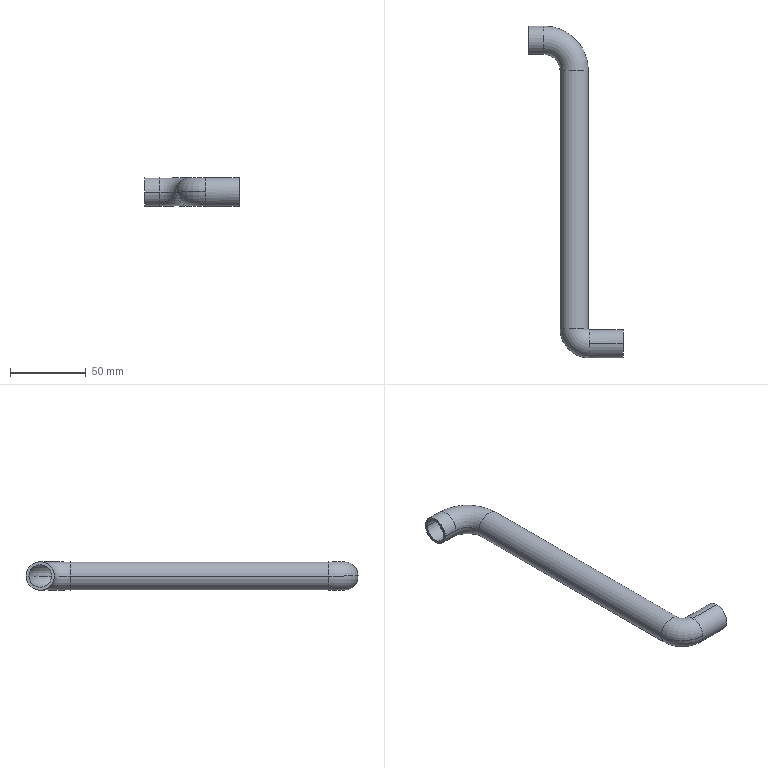Component | SolidWorks | PipeOne-1 | 1 solid | 22 faces | box 62.38 x 219.59 x 18.77 mm | volume 25031 mm3 | cylinder 12 | torus 8 | plane 2 | commonest cylinder face diameters 15 x6 18.77 x6
build123d program:
from build123d import *

# Parameters (mm, degrees)
SKETCH1_R   = 9.385
SKETCH1_R_2 = 7.5


with BuildPart() as part:
    # Sweep5: sweep along a path in Sketch3
    with BuildLine(Plane(origin=(0, 0, 0), x_dir=(0, 0, -1), z_dir=(1, 0, 0))) as sweep5_path:
        Line((0, 0), (-10, 0))
        ThreePointArc((-10, 0), (-24.142, -5.858), (-30, -20))
        Line((-30, -20), (-30, -190.823))
        ThreePointArc((-30, -190.823), (-32.929, -197.894), (-40, -200.823))
        Line((-40, -200.823), (-62.38, -200.823))
    # Sketch1 → Sweep5 (sweep)
    with BuildSketch(Plane.XY):
        Circle(SKETCH1_R)
        Circle(SKETCH1_R_2, mode=Mode.SUBTRACT)
    sweep(path=sweep5_path.line)


solid = part.part

# Placed as in the assembly
solid = solid.moved(Location((598.89, 510.198, -117.25), (0, 90, 0)))
STEP:
#1=CARTESIAN_POINT('',(25.055,12.574,-4.616));
#2=VERTEX_POINT('',#1);
#3=CARTESIAN_POINT('',(24.464,12.574,-4.616));
#4=VERTEX_POINT('',#3);
#5=CARTESIAN_POINT('',(24.759,12.574,-4.616));
#6=DIRECTION('',(-0.,1.,-0.));
#7=DIRECTION('',(0.,0.,-1.));
#8=AXIS2_PLACEMENT_3D('',#5,#6,#7);
#9=CIRCLE('',#8,0.2953);
#10=EDGE_CURVE('',#2,#4,#9,.T.);
#11=ORIENTED_EDGE('',*,*,#10,.T.);
#12=CARTESIAN_POINT('',(25.153,11.885,-4.616));
#13=VERTEX_POINT('',#12);
#14=CARTESIAN_POINT('',(25.153,12.574,-4.616));
#15=DIRECTION('',(-0.,0.,1.));
#16=DIRECTION('',(0.,-1.,0.));
#17=AXIS2_PLACEMENT_3D('',#14,#15,#16);
#18=CIRCLE('',#17,0.689);
#19=EDGE_CURVE('',#4,#13,#18,.T.);
#20=ORIENTED_EDGE('',*,*,#19,.T.);
#21=CARTESIAN_POINT('',(25.153,12.18,-4.911));
#22=VERTEX_POINT('',#21);
#23=CARTESIAN_POINT('',(25.153,12.18,-4.616));
#24=DIRECTION('',(-1.,-0.,-0.));
#25=DIRECTION('',(0.,-0.,-1.));
#26=AXIS2_PLACEMENT_3D('',#23,#24,#25);
#27=CIRCLE('',#26,0.2953);
#28=EDGE_CURVE('',#22,#13,#27,.T.);
#29=ORIENTED_EDGE('',*,*,#28,.F.);
#30=CARTESIAN_POINT('',(25.153,12.475,-4.616));
#31=VERTEX_POINT('',#30);
#32=CARTESIAN_POINT('',(25.153,12.18,-4.616));
#33=DIRECTION('',(-1.,-0.,-0.));
#34=DIRECTION('',(0.,-0.,-1.));
#35=AXIS2_PLACEMENT_3D('',#32,#33,#34);
#36=CIRCLE('',#35,0.2953);
#37=EDGE_CURVE('',#31,#22,#36,.T.);
#38=ORIENTED_EDGE('',*,*,#37,.F.);
#39=CARTESIAN_POINT('',(25.153,12.574,-4.616));
#40=DIRECTION('',(-0.,0.,1.));
#41=DIRECTION('',(0.,-1.,0.));
#42=AXIS2_PLACEMENT_3D('',#39,#40,#41);
#43=CIRCLE('',#42,0.09843);
#44=EDGE_CURVE('',#2,#31,#43,.T.);
#45=ORIENTED_EDGE('',*,*,#44,.F.);
#46=EDGE_LOOP('',(#11,#20,#29,#38,#45));
#47=FACE_OUTER_BOUND('',#46,.T.);
#48=CARTESIAN_POINT('',(25.153,12.574,-4.616));
#49=DIRECTION('',(-0.,0.,1.));
#50=DIRECTION('',(1.,0.,0.));
#51=AXIS2_PLACEMENT_3D('',#48,#49,#50);
#52=TOROIDAL_SURFACE('',#51,0.3937,0.2953);
#53=ADVANCED_FACE('',(#47),#52,.F.);
#54=CARTESIAN_POINT('',(23.972,19.791,-4.616));
#55=VERTEX_POINT('',#54);
#56=CARTESIAN_POINT('',(23.972,20.382,-4.616));
#57=VERTEX_POINT('',#56);
#58=CARTESIAN_POINT('',(23.972,20.087,-4.616));
#59=DIRECTION('',(-1.,-0.,-0.));
#60=DIRECTION('',(0.,0.,-1.));
#61=AXIS2_PLACEMENT_3D('',#58,#59,#60);
#62=CIRCLE('',#61,0.2953);
#63=EDGE_CURVE('',#55,#57,#62,.T.);
#64=ORIENTED_EDGE('',*,*,#63,.T.);
#65=CARTESIAN_POINT('',(25.055,19.299,-4.616));
#66=VERTEX_POINT('',#65);
#67=CARTESIAN_POINT('',(23.972,19.299,-4.616));
#68=DIRECTION('',(0.,-0.,-1.));
#69=DIRECTION('',(0.,1.,-0.));
#70=AXIS2_PLACEMENT_3D('',#67,#68,#69);
#71=CIRCLE('',#70,1.083);
#72=EDGE_CURVE('',#57,#66,#71,.T.);
#73=ORIENTED_EDGE('',*,*,#72,.T.);
#74=CARTESIAN_POINT('',(24.464,19.299,-4.616));
#75=VERTEX_POINT('',#74);
#76=CARTESIAN_POINT('',(24.759,19.299,-4.616));
#77=DIRECTION('',(-0.,1.,-0.));
#78=DIRECTION('',(0.,0.,-1.));
#79=AXIS2_PLACEMENT_3D('',#76,#77,#78);
#80=CIRCLE('',#79,0.2953);
#81=EDGE_CURVE('',#75,#66,#80,.T.);
#82=ORIENTED_EDGE('',*,*,#81,.F.);
#83=CARTESIAN_POINT('',(23.972,19.299,-4.616));
#84=DIRECTION('',(0.,-0.,-1.));
#85=DIRECTION('',(0.,1.,-0.));
#86=AXIS2_PLACEMENT_3D('',#83,#84,#85);
#87=CIRCLE('',#86,0.4921);
#88=EDGE_CURVE('',#55,#75,#87,.T.);
#89=ORIENTED_EDGE('',*,*,#88,.F.);
#90=EDGE_LOOP('',(#64,#73,#82,#89));
#91=FACE_OUTER_BOUND('',#90,.T.);
#92=CARTESIAN_POINT('',(23.972,19.299,-4.616));
#93=DIRECTION('',(0.,-0.,-1.));
#94=DIRECTION('',(-1.,-0.,-0.));
#95=AXIS2_PLACEMENT_3D('',#92,#93,#94);
#96=TOROIDAL_SURFACE('',#95,0.7874,0.2953);
#97=ADVANCED_FACE('',(#91),#96,.F.);
#98=CARTESIAN_POINT('',(25.129,12.574,-4.616));
#99=VERTEX_POINT('',#98);
#100=CARTESIAN_POINT('',(24.39,12.574,-4.616));
#101=VERTEX_POINT('',#100);
#102=CARTESIAN_POINT('',(24.759,12.574,-4.616));
#103=DIRECTION('',(0.,-1.,0.));
#104=DIRECTION('',(0.,-0.,-1.));
#105=AXIS2_PLACEMENT_3D('',#102,#103,#104);
#106=CIRCLE('',#105,0.3695);
#107=EDGE_CURVE('',#99,#101,#106,.T.);
#108=ORIENTED_EDGE('',*,*,#107,.T.);
#109=CARTESIAN_POINT('',(25.153,11.811,-4.616));
#110=VERTEX_POINT('',#109);
#111=CARTESIAN_POINT('',(25.153,12.574,-4.616));
#112=DIRECTION('',(-0.,0.,1.));
#113=DIRECTION('',(0.,-1.,0.));
#114=AXIS2_PLACEMENT_3D('',#111,#112,#113);
#115=CIRCLE('',#114,0.7632);
#116=EDGE_CURVE('',#101,#110,#115,.T.);
#117=ORIENTED_EDGE('',*,*,#116,.T.);
#118=CARTESIAN_POINT('',(25.153,12.18,-4.247));
#119=VERTEX_POINT('',#118);
#120=CARTESIAN_POINT('',(25.153,12.18,-4.616));
#121=DIRECTION('',(1.,0.,0.));
#122=DIRECTION('',(0.,-0.,-1.));
#123=AXIS2_PLACEMENT_3D('',#120,#121,#122);
#124=CIRCLE('',#123,0.3695);
#125=EDGE_CURVE('',#119,#110,#124,.T.);
#126=ORIENTED_EDGE('',*,*,#125,.F.);
#127=CARTESIAN_POINT('',(25.153,12.55,-4.616));
#128=VERTEX_POINT('',#127);
#129=CARTESIAN_POINT('',(25.153,12.18,-4.616));
#130=DIRECTION('',(1.,0.,0.));
#131=DIRECTION('',(0.,-0.,-1.));
#132=AXIS2_PLACEMENT_3D('',#129,#130,#131);
#133=CIRCLE('',#132,0.3695);
#134=EDGE_CURVE('',#128,#119,#133,.T.);
#135=ORIENTED_EDGE('',*,*,#134,.F.);
#136=CARTESIAN_POINT('',(25.153,12.574,-4.616));
#137=DIRECTION('',(-0.,0.,1.));
#138=DIRECTION('',(0.,-1.,0.));
#139=AXIS2_PLACEMENT_3D('',#136,#137,#138);
#140=CIRCLE('',#139,0.02421);
#141=EDGE_CURVE('',#99,#128,#140,.T.);
#142=ORIENTED_EDGE('',*,*,#141,.F.);
#143=EDGE_LOOP('',(#108,#117,#126,#135,#142));
#144=FACE_OUTER_BOUND('',#143,.T.);
#145=CARTESIAN_POINT('',(25.153,12.574,-4.616));
#146=DIRECTION('',(-0.,0.,1.));
#147=DIRECTION('',(1.,0.,0.));
#148=AXIS2_PLACEMENT_3D('',#145,#146,#147);
#149=TOROIDAL_SURFACE('',#148,0.3937,0.3695);
#150=ADVANCED_FACE('',(#144),#149,.T.);
#151=CARTESIAN_POINT('',(23.972,19.717,-4.616));
#152=VERTEX_POINT('',#151);
#153=CARTESIAN_POINT('',(23.972,20.456,-4.616));
#154=VERTEX_POINT('',#153);
#155=CARTESIAN_POINT('',(23.972,20.087,-4.616));
#156=DIRECTION('',(1.,0.,0.));
#157=DIRECTION('',(0.,0.,-1.));
#158=AXIS2_PLACEMENT_3D('',#155,#156,#157);
#159=CIRCLE('',#158,0.3695);
#160=EDGE_CURVE('',#152,#154,#159,.T.);
#161=ORIENTED_EDGE('',*,*,#160,.T.);
#162=CARTESIAN_POINT('',(25.129,19.299,-4.616));
#163=VERTEX_POINT('',#162);
#164=CARTESIAN_POINT('',(23.972,19.299,-4.616));
#165=DIRECTION('',(0.,-0.,-1.));
#166=DIRECTION('',(0.,1.,-0.));
#167=AXIS2_PLACEMENT_3D('',#164,#165,#166);
#168=CIRCLE('',#167,1.157);
#169=EDGE_CURVE('',#154,#163,#168,.T.);
#170=ORIENTED_EDGE('',*,*,#169,.T.);
#171=CARTESIAN_POINT('',(24.39,19.299,-4.616));
#172=VERTEX_POINT('',#171);
#173=CARTESIAN_POINT('',(24.759,19.299,-4.616));
#174=DIRECTION('',(0.,-1.,0.));
#175=DIRECTION('',(0.,-0.,-1.));
#176=AXIS2_PLACEMENT_3D('',#173,#174,#175);
#177=CIRCLE('',#176,0.3695);
#178=EDGE_CURVE('',#172,#163,#177,.T.);
#179=ORIENTED_EDGE('',*,*,#178,.F.);
#180=CARTESIAN_POINT('',(23.972,19.299,-4.616));
#181=DIRECTION('',(0.,-0.,-1.));
#182=DIRECTION('',(0.,1.,-0.));
#183=AXIS2_PLACEMENT_3D('',#180,#181,#182);
#184=CIRCLE('',#183,0.4179);
#185=EDGE_CURVE('',#152,#172,#184,.T.);
#186=ORIENTED_EDGE('',*,*,#185,.F.);
#187=EDGE_LOOP('',(#161,#170,#179,#186));
#188=FACE_OUTER_BOUND('',#187,.T.);
#189=CARTESIAN_POINT('',(23.972,19.299,-4.616));
#190=DIRECTION('',(0.,-0.,-1.));
#191=DIRECTION('',(-1.,-0.,-0.));
#192=AXIS2_PLACEMENT_3D('',#189,#190,#191);
#193=TOROIDAL_SURFACE('',#192,0.7874,0.3695);
#194=ADVANCED_FACE('',(#188),#193,.T.);
#195=ORIENTED_EDGE('',*,*,#28,.T.);
#196=CARTESIAN_POINT('',(25.153,12.18,-4.321));
#197=VERTEX_POINT('',#196);
#198=CARTESIAN_POINT('',(25.153,12.18,-4.616));
#199=DIRECTION('',(-1.,-0.,-0.));
#200=DIRECTION('',(0.,0.,-1.));
#201=AXIS2_PLACEMENT_3D('',#198,#199,#200);
#202=CIRCLE('',#201,0.2953);
#203=EDGE_CURVE('',#13,#197,#202,.T.);
#204=ORIENTED_EDGE('',*,*,#203,.T.);
#205=CARTESIAN_POINT('',(26.034,12.18,-4.321));
#206=VERTEX_POINT('',#205);
#207=CARTESIAN_POINT('',(25.153,12.18,-4.321));
#208=DIRECTION('',(1.,0.,0.));
#209=VECTOR('',#208,39.37);
#210=LINE('',#207,#209);
#211=EDGE_CURVE('',#197,#206,#210,.T.);
#212=ORIENTED_EDGE('',*,*,#211,.T.);
#213=CARTESIAN_POINT('',(26.034,12.18,-4.911));
#214=VERTEX_POINT('',#213);
#215=CARTESIAN_POINT('',(26.034,12.18,-4.616));
#216=DIRECTION('',(-1.,-0.,-0.));
#217=DIRECTION('',(0.,-0.,-1.));
#218=AXIS2_PLACEMENT_3D('',#215,#216,#217);
#219=CIRCLE('',#218,0.2953);
#220=EDGE_CURVE('',#214,#206,#219,.T.);
#221=ORIENTED_EDGE('',*,*,#220,.F.);
#222=CARTESIAN_POINT('',(25.153,12.18,-4.911));
#223=DIRECTION('',(1.,0.,0.));
#224=VECTOR('',#223,39.37);
#225=LINE('',#222,#224);
#226=EDGE_CURVE('',#22,#214,#225,.T.);
#227=ORIENTED_EDGE('',*,*,#226,.F.);
#228=EDGE_LOOP('',(#195,#204,#212,#221,#227));
#229=FACE_OUTER_BOUND('',#228,.T.);
#230=CARTESIAN_POINT('',(25.153,12.18,-4.616));
#231=DIRECTION('',(1.,0.,0.));
#232=DIRECTION('',(0.,0.,-1.));
#233=AXIS2_PLACEMENT_3D('',#230,#231,#232);
#234=CYLINDRICAL_SURFACE('',#233,0.2953);
#235=ADVANCED_FACE('',(#229),#234,.F.);
#236=ORIENTED_EDGE('',*,*,#81,.T.);
#237=CARTESIAN_POINT('',(25.055,19.299,-4.616));
#238=DIRECTION('',(0.,-1.,0.));
#239=VECTOR('',#238,39.37);
#240=LINE('',#237,#239);
#241=EDGE_CURVE('',#66,#2,#240,.T.);
#242=ORIENTED_EDGE('',*,*,#241,.T.);
#243=CARTESIAN_POINT('',(24.759,12.574,-4.616));
#244=DIRECTION('',(-0.,1.,-0.));
#245=DIRECTION('',(0.,0.,-1.));
#246=AXIS2_PLACEMENT_3D('',#243,#244,#245);
#247=CIRCLE('',#246,0.2953);
#248=EDGE_CURVE('',#4,#2,#247,.T.);
#249=ORIENTED_EDGE('',*,*,#248,.F.);
#250=CARTESIAN_POINT('',(24.464,19.299,-4.616));
#251=DIRECTION('',(0.,-1.,0.));
#252=VECTOR('',#251,39.37);
#253=LINE('',#250,#252);
#254=EDGE_CURVE('',#75,#4,#253,.T.);
#255=ORIENTED_EDGE('',*,*,#254,.F.);
#256=EDGE_LOOP('',(#236,#242,#249,#255));
#257=FACE_OUTER_BOUND('',#256,.T.);
#258=CARTESIAN_POINT('',(24.759,19.299,-4.616));
#259=DIRECTION('',(0.,-1.,0.));
#260=DIRECTION('',(-1.,0.,0.));
#261=AXIS2_PLACEMENT_3D('',#258,#259,#260);
#262=CYLINDRICAL_SURFACE('',#261,0.2953);
#263=ADVANCED_FACE('',(#257),#262,.F.);
#264=CARTESIAN_POINT('',(23.578,19.791,-4.616));
#265=VERTEX_POINT('',#264);
#266=CARTESIAN_POINT('',(23.578,20.382,-4.616));
#267=VERTEX_POINT('',#266);
#268=CARTESIAN_POINT('',(23.578,20.087,-4.616));
#269=DIRECTION('',(-1.,-0.,-0.));
#270=DIRECTION('',(0.,0.,-1.));
#271=AXIS2_PLACEMENT_3D('',#268,#269,#270);
#272=CIRCLE('',#271,0.2953);
#273=EDGE_CURVE('',#265,#267,#272,.T.);
#274=ORIENTED_EDGE('',*,*,#273,.T.);
#275=CARTESIAN_POINT('',(23.578,20.382,-4.616));
#276=DIRECTION('',(1.,0.,0.));
#277=VECTOR('',#276,39.37);
#278=LINE('',#275,#277);
#279=EDGE_CURVE('',#267,#57,#278,.T.);
#280=ORIENTED_EDGE('',*,*,#279,.T.);
#281=ORIENTED_EDGE('',*,*,#63,.F.);
#282=CARTESIAN_POINT('',(23.578,19.791,-4.616));
#283=DIRECTION('',(1.,0.,0.));
#284=VECTOR('',#283,39.37);
#285=LINE('',#282,#284);
#286=EDGE_CURVE('',#265,#55,#285,.T.);
#287=ORIENTED_EDGE('',*,*,#286,.F.);
#288=EDGE_LOOP('',(#274,#280,#281,#287));
#289=FACE_OUTER_BOUND('',#288,.T.);
#290=CARTESIAN_POINT('',(23.578,20.087,-4.616));
#291=DIRECTION('',(1.,0.,0.));
#292=DIRECTION('',(0.,-1.,0.));
#293=AXIS2_PLACEMENT_3D('',#290,#291,#292);
#294=CYLINDRICAL_SURFACE('',#293,0.2953);
#295=ADVANCED_FACE('',(#289),#294,.F.);
#296=CARTESIAN_POINT('',(25.153,12.18,-4.986));
#297=VERTEX_POINT('',#296);
#298=CARTESIAN_POINT('',(25.153,12.18,-4.616));
#299=DIRECTION('',(1.,0.,0.));
#300=DIRECTION('',(0.,-0.,-1.));
#301=AXIS2_PLACEMENT_3D('',#298,#299,#300);
#302=CIRCLE('',#301,0.3695);
#303=EDGE_CURVE('',#297,#128,#302,.T.);
#304=ORIENTED_EDGE('',*,*,#303,.T.);
#305=ORIENTED_EDGE('',*,*,#134,.T.);
#306=CARTESIAN_POINT('',(26.034,12.18,-4.247));
#307=VERTEX_POINT('',#306);
#308=CARTESIAN_POINT('',(25.153,12.18,-4.247));
#309=DIRECTION('',(1.,0.,0.));
#310=VECTOR('',#309,39.37);
#311=LINE('',#308,#310);
#312=EDGE_CURVE('',#119,#307,#311,.T.);
#313=ORIENTED_EDGE('',*,*,#312,.T.);
#314=CARTESIAN_POINT('',(26.034,12.18,-4.986));
#315=VERTEX_POINT('',#314);
#316=CARTESIAN_POINT('',(26.034,12.18,-4.616));
#317=DIRECTION('',(1.,0.,0.));
#318=DIRECTION('',(0.,-0.,-1.));
#319=AXIS2_PLACEMENT_3D('',#316,#317,#318);
#320=CIRCLE('',#319,0.3695);
#321=EDGE_CURVE('',#315,#307,#320,.T.);
#322=ORIENTED_EDGE('',*,*,#321,.F.);
#323=CARTESIAN_POINT('',(25.153,12.18,-4.986));
#324=DIRECTION('',(1.,0.,0.));
#325=VECTOR('',#324,39.37);
#326=LINE('',#323,#325);
#327=EDGE_CURVE('',#297,#315,#326,.T.);
#328=ORIENTED_EDGE('',*,*,#327,.F.);
#329=EDGE_LOOP('',(#304,#305,#313,#322,#328));
#330=FACE_OUTER_BOUND('',#329,.T.);
#331=CARTESIAN_POINT('',(25.153,12.18,-4.616));
#332=DIRECTION('',(1.,0.,0.));
#333=DIRECTION('',(0.,-0.,-1.));
#334=AXIS2_PLACEMENT_3D('',#331,#332,#333);
#335=CYLINDRICAL_SURFACE('',#334,0.3695);
#336=ADVANCED_FACE('',(#330),#335,.T.);
#337=ORIENTED_EDGE('',*,*,#178,.T.);
#338=CARTESIAN_POINT('',(25.129,19.299,-4.616));
#339=DIRECTION('',(0.,-1.,0.));
#340=VECTOR('',#339,39.37);
#341=LINE('',#338,#340);
#342=EDGE_CURVE('',#163,#99,#341,.T.);
#343=ORIENTED_EDGE('',*,*,#342,.T.);
#344=CARTESIAN_POINT('',(24.759,12.574,-4.616));
#345=DIRECTION('',(0.,-1.,0.));
#346=DIRECTION('',(0.,-0.,-1.));
#347=AXIS2_PLACEMENT_3D('',#344,#345,#346);
#348=CIRCLE('',#347,0.3695);
#349=EDGE_CURVE('',#101,#99,#348,.T.);
#350=ORIENTED_EDGE('',*,*,#349,.F.);
#351=CARTESIAN_POINT('',(24.39,19.299,-4.616));
#352=DIRECTION('',(0.,-1.,0.));
#353=VECTOR('',#352,39.37);
#354=LINE('',#351,#353);
#355=EDGE_CURVE('',#172,#101,#354,.T.);
#356=ORIENTED_EDGE('',*,*,#355,.F.);
#357=EDGE_LOOP('',(#337,#343,#350,#356));
#358=FACE_OUTER_BOUND('',#357,.T.);
#359=CARTESIAN_POINT('',(24.759,19.299,-4.616));
#360=DIRECTION('',(0.,-1.,0.));
#361=DIRECTION('',(-1.,-0.,0.));
#362=AXIS2_PLACEMENT_3D('',#359,#360,#361);
#363=CYLINDRICAL_SURFACE('',#362,0.3695);
#364=ADVANCED_FACE('',(#358),#363,.T.);
#365=CARTESIAN_POINT('',(23.578,19.717,-4.616));
#366=VERTEX_POINT('',#365);
#367=CARTESIAN_POINT('',(23.578,20.456,-4.616));
#368=VERTEX_POINT('',#367);
#369=CARTESIAN_POINT('',(23.578,20.087,-4.616));
#370=DIRECTION('',(1.,0.,0.));
#371=DIRECTION('',(0.,0.,-1.));
#372=AXIS2_PLACEMENT_3D('',#369,#370,#371);
#373=CIRCLE('',#372,0.3695);
#374=EDGE_CURVE('',#366,#368,#373,.T.);
#375=ORIENTED_EDGE('',*,*,#374,.T.);
#376=CARTESIAN_POINT('',(23.578,20.456,-4.616));
#377=DIRECTION('',(1.,0.,0.));
#378=VECTOR('',#377,39.37);
#379=LINE('',#376,#378);
#380=EDGE_CURVE('',#368,#154,#379,.T.);
#381=ORIENTED_EDGE('',*,*,#380,.T.);
#382=ORIENTED_EDGE('',*,*,#160,.F.);
#383=CARTESIAN_POINT('',(23.578,19.717,-4.616));
#384=DIRECTION('',(1.,0.,0.));
#385=VECTOR('',#384,39.37);
#386=LINE('',#383,#385);
#387=EDGE_CURVE('',#366,#152,#386,.T.);
#388=ORIENTED_EDGE('',*,*,#387,.F.);
#389=EDGE_LOOP('',(#375,#381,#382,#388));
#390=FACE_OUTER_BOUND('',#389,.T.);
#391=CARTESIAN_POINT('',(23.578,20.087,-4.616));
#392=DIRECTION('',(1.,0.,0.));
#393=DIRECTION('',(0.,-1.,0.));
#394=AXIS2_PLACEMENT_3D('',#391,#392,#393);
#395=CYLINDRICAL_SURFACE('',#394,0.3695);
#396=ADVANCED_FACE('',(#390),#395,.T.);
#397=ORIENTED_EDGE('',*,*,#211,.F.);
#398=CARTESIAN_POINT('',(25.153,12.18,-4.616));
#399=DIRECTION('',(-1.,-0.,-0.));
#400=DIRECTION('',(0.,0.,-1.));
#401=AXIS2_PLACEMENT_3D('',#398,#399,#400);
#402=CIRCLE('',#401,0.2953);
#403=EDGE_CURVE('',#197,#31,#402,.T.);
#404=ORIENTED_EDGE('',*,*,#403,.T.);
#405=ORIENTED_EDGE('',*,*,#37,.T.);
#406=ORIENTED_EDGE('',*,*,#226,.T.);
#407=CARTESIAN_POINT('',(26.034,12.18,-4.616));
#408=DIRECTION('',(-1.,-0.,-0.));
#409=DIRECTION('',(0.,-0.,-1.));
#410=AXIS2_PLACEMENT_3D('',#407,#408,#409);
#411=CIRCLE('',#410,0.2953);
#412=EDGE_CURVE('',#206,#214,#411,.T.);
#413=ORIENTED_EDGE('',*,*,#412,.F.);
#414=EDGE_LOOP('',(#397,#404,#405,#406,#413));
#415=FACE_OUTER_BOUND('',#414,.T.);
#416=CARTESIAN_POINT('',(25.153,12.18,-4.616));
#417=DIRECTION('',(1.,0.,0.));
#418=DIRECTION('',(0.,0.,-1.));
#419=AXIS2_PLACEMENT_3D('',#416,#417,#418);
#420=CYLINDRICAL_SURFACE('',#419,0.2953);
#421=ADVANCED_FACE('',(#415),#420,.F.);
#422=ORIENTED_EDGE('',*,*,#19,.F.);
#423=ORIENTED_EDGE('',*,*,#248,.T.);
#424=ORIENTED_EDGE('',*,*,#44,.T.);
#425=ORIENTED_EDGE('',*,*,#403,.F.);
#426=ORIENTED_EDGE('',*,*,#203,.F.);
#427=EDGE_LOOP('',(#422,#423,#424,#425,#426));
#428=FACE_OUTER_BOUND('',#427,.T.);
#429=CARTESIAN_POINT('',(25.153,12.574,-4.616));
#430=DIRECTION('',(-0.,0.,1.));
#431=DIRECTION('',(1.,0.,0.));
#432=AXIS2_PLACEMENT_3D('',#429,#430,#431);
#433=TOROIDAL_SURFACE('',#432,0.3937,0.2953);
#434=ADVANCED_FACE('',(#428),#433,.F.);
#435=ORIENTED_EDGE('',*,*,#241,.F.);
#436=CARTESIAN_POINT('',(24.759,19.299,-4.616));
#437=DIRECTION('',(-0.,1.,-0.));
#438=DIRECTION('',(0.,0.,-1.));
#439=AXIS2_PLACEMENT_3D('',#436,#437,#438);
#440=CIRCLE('',#439,0.2953);
#441=EDGE_CURVE('',#66,#75,#440,.T.);
#442=ORIENTED_EDGE('',*,*,#441,.T.);
#443=ORIENTED_EDGE('',*,*,#254,.T.);
#444=ORIENTED_EDGE('',*,*,#10,.F.);
#445=EDGE_LOOP('',(#435,#442,#443,#444));
#446=FACE_OUTER_BOUND('',#445,.T.);
#447=CARTESIAN_POINT('',(24.759,19.299,-4.616));
#448=DIRECTION('',(0.,-1.,0.));
#449=DIRECTION('',(-1.,0.,0.));
#450=AXIS2_PLACEMENT_3D('',#447,#448,#449);
#451=CYLINDRICAL_SURFACE('',#450,0.2953);
#452=ADVANCED_FACE('',(#446),#451,.F.);
#453=ORIENTED_EDGE('',*,*,#72,.F.);
#454=CARTESIAN_POINT('',(23.972,20.087,-4.616));
#455=DIRECTION('',(-1.,-0.,-0.));
#456=DIRECTION('',(0.,0.,-1.));
#457=AXIS2_PLACEMENT_3D('',#454,#455,#456);
#458=CIRCLE('',#457,0.2953);
#459=EDGE_CURVE('',#57,#55,#458,.T.);
#460=ORIENTED_EDGE('',*,*,#459,.T.);
#461=ORIENTED_EDGE('',*,*,#88,.T.);
#462=ORIENTED_EDGE('',*,*,#441,.F.);
#463=EDGE_LOOP('',(#453,#460,#461,#462));
#464=FACE_OUTER_BOUND('',#463,.T.);
#465=CARTESIAN_POINT('',(23.972,19.299,-4.616));
#466=DIRECTION('',(0.,-0.,-1.));
#467=DIRECTION('',(-1.,-0.,-0.));
#468=AXIS2_PLACEMENT_3D('',#465,#466,#467);
#469=TOROIDAL_SURFACE('',#468,0.7874,0.2953);
#470=ADVANCED_FACE('',(#464),#469,.F.);
#471=ORIENTED_EDGE('',*,*,#279,.F.);
#472=CARTESIAN_POINT('',(23.578,20.087,-4.616));
#473=DIRECTION('',(-1.,-0.,-0.));
#474=DIRECTION('',(0.,0.,-1.));
#475=AXIS2_PLACEMENT_3D('',#472,#473,#474);
#476=CIRCLE('',#475,0.2953);
#477=EDGE_CURVE('',#267,#265,#476,.T.);
#478=ORIENTED_EDGE('',*,*,#477,.T.);
#479=ORIENTED_EDGE('',*,*,#286,.T.);
#480=ORIENTED_EDGE('',*,*,#459,.F.);
#481=EDGE_LOOP('',(#471,#478,#479,#480));
#482=FACE_OUTER_BOUND('',#481,.T.);
#483=CARTESIAN_POINT('',(23.578,20.087,-4.616));
#484=DIRECTION('',(1.,0.,0.));
#485=DIRECTION('',(0.,-1.,0.));
#486=AXIS2_PLACEMENT_3D('',#483,#484,#485);
#487=CYLINDRICAL_SURFACE('',#486,0.2953);
#488=ADVANCED_FACE('',(#482),#487,.F.);
#489=ORIENTED_EDGE('',*,*,#220,.T.);
#490=ORIENTED_EDGE('',*,*,#412,.T.);
#491=EDGE_LOOP('',(#489,#490));
#492=FACE_BOUND('',#491,.T.);
#493=ORIENTED_EDGE('',*,*,#321,.T.);
#494=CARTESIAN_POINT('',(26.034,12.18,-4.616));
#495=DIRECTION('',(1.,0.,0.));
#496=DIRECTION('',(0.,-0.,-1.));
#497=AXIS2_PLACEMENT_3D('',#494,#495,#496);
#498=CIRCLE('',#497,0.3695);
#499=EDGE_CURVE('',#307,#315,#498,.T.);
#500=ORIENTED_EDGE('',*,*,#499,.T.);
#501=EDGE_LOOP('',(#493,#500));
#502=FACE_OUTER_BOUND('',#501,.T.);
#503=CARTESIAN_POINT('',(26.034,12.18,-4.616));
#504=DIRECTION('',(1.,0.,0.));
#505=DIRECTION('',(0.,-0.,-1.));
#506=AXIS2_PLACEMENT_3D('',#503,#504,#505);
#507=PLANE('',#506);
#508=ADVANCED_FACE('',(#492,#502),#507,.T.);
#509=ORIENTED_EDGE('',*,*,#273,.F.);
#510=ORIENTED_EDGE('',*,*,#477,.F.);
#511=EDGE_LOOP('',(#509,#510));
#512=FACE_BOUND('',#511,.T.);
#513=ORIENTED_EDGE('',*,*,#374,.F.);
#514=CARTESIAN_POINT('',(23.578,20.087,-4.616));
#515=DIRECTION('',(1.,0.,0.));
#516=DIRECTION('',(0.,0.,-1.));
#517=AXIS2_PLACEMENT_3D('',#514,#515,#516);
#518=CIRCLE('',#517,0.3695);
#519=EDGE_CURVE('',#368,#366,#518,.T.);
#520=ORIENTED_EDGE('',*,*,#519,.F.);
#521=EDGE_LOOP('',(#513,#520));
#522=FACE_OUTER_BOUND('',#521,.T.);
#523=CARTESIAN_POINT('',(23.578,20.087,-4.616));
#524=DIRECTION('',(1.,0.,0.));
#525=DIRECTION('',(0.,-0.,-1.));
#526=AXIS2_PLACEMENT_3D('',#523,#524,#525);
#527=PLANE('',#526);
#528=ADVANCED_FACE('',(#512,#522),#527,.F.);
#529=ORIENTED_EDGE('',*,*,#312,.F.);
#530=ORIENTED_EDGE('',*,*,#125,.T.);
#531=CARTESIAN_POINT('',(25.153,12.18,-4.616));
#532=DIRECTION('',(1.,0.,0.));
#533=DIRECTION('',(0.,-0.,-1.));
#534=AXIS2_PLACEMENT_3D('',#531,#532,#533);
#535=CIRCLE('',#534,0.3695);
#536=EDGE_CURVE('',#110,#297,#535,.T.);
#537=ORIENTED_EDGE('',*,*,#536,.T.);
#538=ORIENTED_EDGE('',*,*,#327,.T.);
#539=ORIENTED_EDGE('',*,*,#499,.F.);
#540=EDGE_LOOP('',(#529,#530,#537,#538,#539));
#541=FACE_OUTER_BOUND('',#540,.T.);
#542=CARTESIAN_POINT('',(25.153,12.18,-4.616));
#543=DIRECTION('',(1.,0.,0.));
#544=DIRECTION('',(0.,-0.,-1.));
#545=AXIS2_PLACEMENT_3D('',#542,#543,#544);
#546=CYLINDRICAL_SURFACE('',#545,0.3695);
#547=ADVANCED_FACE('',(#541),#546,.T.);
#548=ORIENTED_EDGE('',*,*,#116,.F.);
#549=ORIENTED_EDGE('',*,*,#349,.T.);
#550=ORIENTED_EDGE('',*,*,#141,.T.);
#551=ORIENTED_EDGE('',*,*,#303,.F.);
#552=ORIENTED_EDGE('',*,*,#536,.F.);
#553=EDGE_LOOP('',(#548,#549,#550,#551,#552));
#554=FACE_OUTER_BOUND('',#553,.T.);
#555=CARTESIAN_POINT('',(25.153,12.574,-4.616));
#556=DIRECTION('',(-0.,0.,1.));
#557=DIRECTION('',(1.,0.,0.));
#558=AXIS2_PLACEMENT_3D('',#555,#556,#557);
#559=TOROIDAL_SURFACE('',#558,0.3937,0.3695);
#560=ADVANCED_FACE('',(#554),#559,.T.);
#561=ORIENTED_EDGE('',*,*,#342,.F.);
#562=CARTESIAN_POINT('',(24.759,19.299,-4.616));
#563=DIRECTION('',(0.,-1.,0.));
#564=DIRECTION('',(0.,-0.,-1.));
#565=AXIS2_PLACEMENT_3D('',#562,#563,#564);
#566=CIRCLE('',#565,0.3695);
#567=EDGE_CURVE('',#163,#172,#566,.T.);
#568=ORIENTED_EDGE('',*,*,#567,.T.);
#569=ORIENTED_EDGE('',*,*,#355,.T.);
#570=ORIENTED_EDGE('',*,*,#107,.F.);
#571=EDGE_LOOP('',(#561,#568,#569,#570));
#572=FACE_OUTER_BOUND('',#571,.T.);
#573=CARTESIAN_POINT('',(24.759,19.299,-4.616));
#574=DIRECTION('',(0.,-1.,0.));
#575=DIRECTION('',(-1.,-0.,0.));
#576=AXIS2_PLACEMENT_3D('',#573,#574,#575);
#577=CYLINDRICAL_SURFACE('',#576,0.3695);
#578=ADVANCED_FACE('',(#572),#577,.T.);
#579=ORIENTED_EDGE('',*,*,#169,.F.);
#580=CARTESIAN_POINT('',(23.972,20.087,-4.616));
#581=DIRECTION('',(1.,0.,0.));
#582=DIRECTION('',(0.,0.,-1.));
#583=AXIS2_PLACEMENT_3D('',#580,#581,#582);
#584=CIRCLE('',#583,0.3695);
#585=EDGE_CURVE('',#154,#152,#584,.T.);
#586=ORIENTED_EDGE('',*,*,#585,.T.);
#587=ORIENTED_EDGE('',*,*,#185,.T.);
#588=ORIENTED_EDGE('',*,*,#567,.F.);
#589=EDGE_LOOP('',(#579,#586,#587,#588));
#590=FACE_OUTER_BOUND('',#589,.T.);
#591=CARTESIAN_POINT('',(23.972,19.299,-4.616));
#592=DIRECTION('',(0.,-0.,-1.));
#593=DIRECTION('',(-1.,-0.,-0.));
#594=AXIS2_PLACEMENT_3D('',#591,#592,#593);
#595=TOROIDAL_SURFACE('',#594,0.7874,0.3695);
#596=ADVANCED_FACE('',(#590),#595,.T.);
#597=ORIENTED_EDGE('',*,*,#380,.F.);
#598=ORIENTED_EDGE('',*,*,#519,.T.);
#599=ORIENTED_EDGE('',*,*,#387,.T.);
#600=ORIENTED_EDGE('',*,*,#585,.F.);
#601=EDGE_LOOP('',(#597,#598,#599,#600));
#602=FACE_OUTER_BOUND('',#601,.T.);
#603=CARTESIAN_POINT('',(23.578,20.087,-4.616));
#604=DIRECTION('',(1.,0.,0.));
#605=DIRECTION('',(0.,-1.,0.));
#606=AXIS2_PLACEMENT_3D('',#603,#604,#605);
#607=CYLINDRICAL_SURFACE('',#606,0.3695);
#608=ADVANCED_FACE('',(#602),#607,.T.);
#609=CLOSED_SHELL('',(#53,#97,#150,#194,#235,#263,#295,#336,#364,#396,#421,#434,#452,#470,#488,#508,#528,#547,#560,#578,#596,#608));
#610=MANIFOLD_SOLID_BREP('',#609);
#611=CARTESIAN_POINT('',(0.,0.,0.));
#612=DIRECTION('',(0.,0.,1.));
#613=DIRECTION('',(1.,0.,0.));
#614=AXIS2_PLACEMENT_3D('',#611,#612,#613);
#615=(LENGTH_UNIT()NAMED_UNIT(*)SI_UNIT($,.METRE.));
#616=LENGTH_MEASURE_WITH_UNIT(LENGTH_MEASURE(0.0254),#615);
#617=DIMENSIONAL_EXPONENTS(1.,0.,0.,0.,0.,0.,0.);
#618=(CONVERSION_BASED_UNIT('',#616)LENGTH_UNIT()NAMED_UNIT(#617));
#619=UNCERTAINTY_MEASURE_WITH_UNIT(LENGTH_MEASURE(0.00001),#618,'','');
#620=(NAMED_UNIT(*)PLANE_ANGLE_UNIT()SI_UNIT($,.RADIAN.));
#621=(NAMED_UNIT(*)SI_UNIT($,.STERADIAN.)SOLID_ANGLE_UNIT());
#622=(GEOMETRIC_REPRESENTATION_CONTEXT(3)GLOBAL_UNCERTAINTY_ASSIGNED_CONTEXT((#619))GLOBAL_UNIT_ASSIGNED_CONTEXT((#618,#620,#621))REPRESENTATION_CONTEXT('',''));
#623=ADVANCED_BREP_SHAPE_REPRESENTATION('',(#610,#614),#622);
#624=COLOUR_RGB('',0.7922,0.8196,0.9333);
#625=FILL_AREA_STYLE_COLOUR('',#624);
#626=FILL_AREA_STYLE('',(#625));
#627=SURFACE_STYLE_FILL_AREA(#626);
#628=SURFACE_SIDE_STYLE('',(#627));
#629=SURFACE_STYLE_USAGE(.BOTH.,#628);
#630=PRESENTATION_STYLE_ASSIGNMENT((#629));
#631=STYLED_ITEM('',(#630),#610);
#632=(LENGTH_UNIT()NAMED_UNIT(*)SI_UNIT($,.METRE.));
#633=LENGTH_MEASURE_WITH_UNIT(LENGTH_MEASURE(0.0254),#632);
#634=DIMENSIONAL_EXPONENTS(1.,0.,0.,0.,0.,0.,0.);
#635=(CONVERSION_BASED_UNIT('',#633)LENGTH_UNIT()NAMED_UNIT(#634));
#636=UNCERTAINTY_MEASURE_WITH_UNIT(LENGTH_MEASURE(0.00001),#635,'','');
#637=(NAMED_UNIT(*)PLANE_ANGLE_UNIT()SI_UNIT($,.RADIAN.));
#638=(NAMED_UNIT(*)SI_UNIT($,.STERADIAN.)SOLID_ANGLE_UNIT());
#639=(GEOMETRIC_REPRESENTATION_CONTEXT(3)GLOBAL_UNCERTAINTY_ASSIGNED_CONTEXT((#636))GLOBAL_UNIT_ASSIGNED_CONTEXT((#635,#637,#638))REPRESENTATION_CONTEXT('',''));
#640=MECHANICAL_DESIGN_GEOMETRIC_PRESENTATION_REPRESENTATION('',(#631),#639);
#641=PRESENTATION_LAYER_ASSIGNMENT('','',(#631));